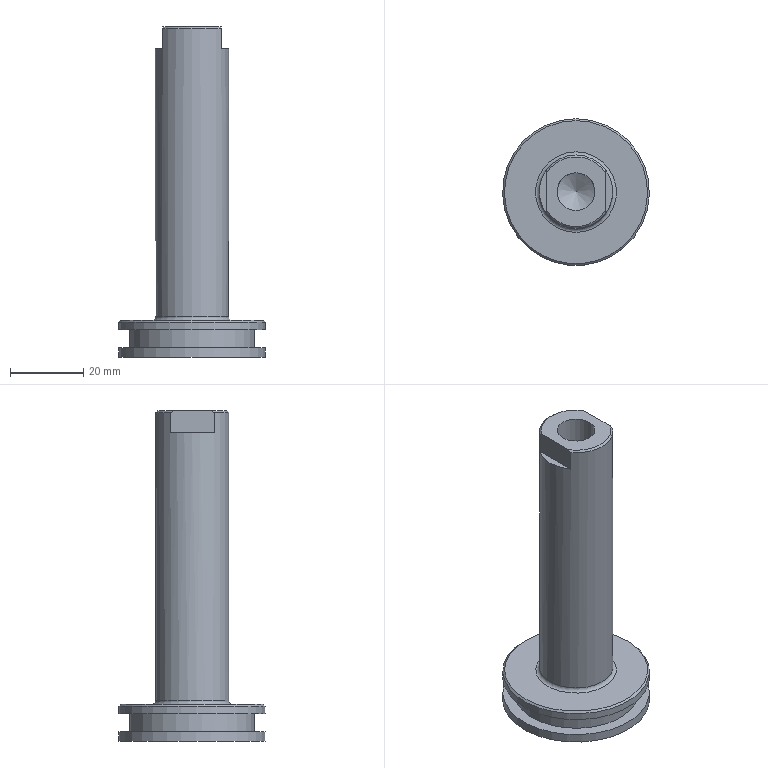Component | NX | PISTON_ROD | 1 solid | 19 faces | volume 34167 mm3 | plane 9 | cylinder 5 | cone 4 | torus 1 | commonest cylinder face diameters 40 x2 20 x1 34 x1 10.3 x1